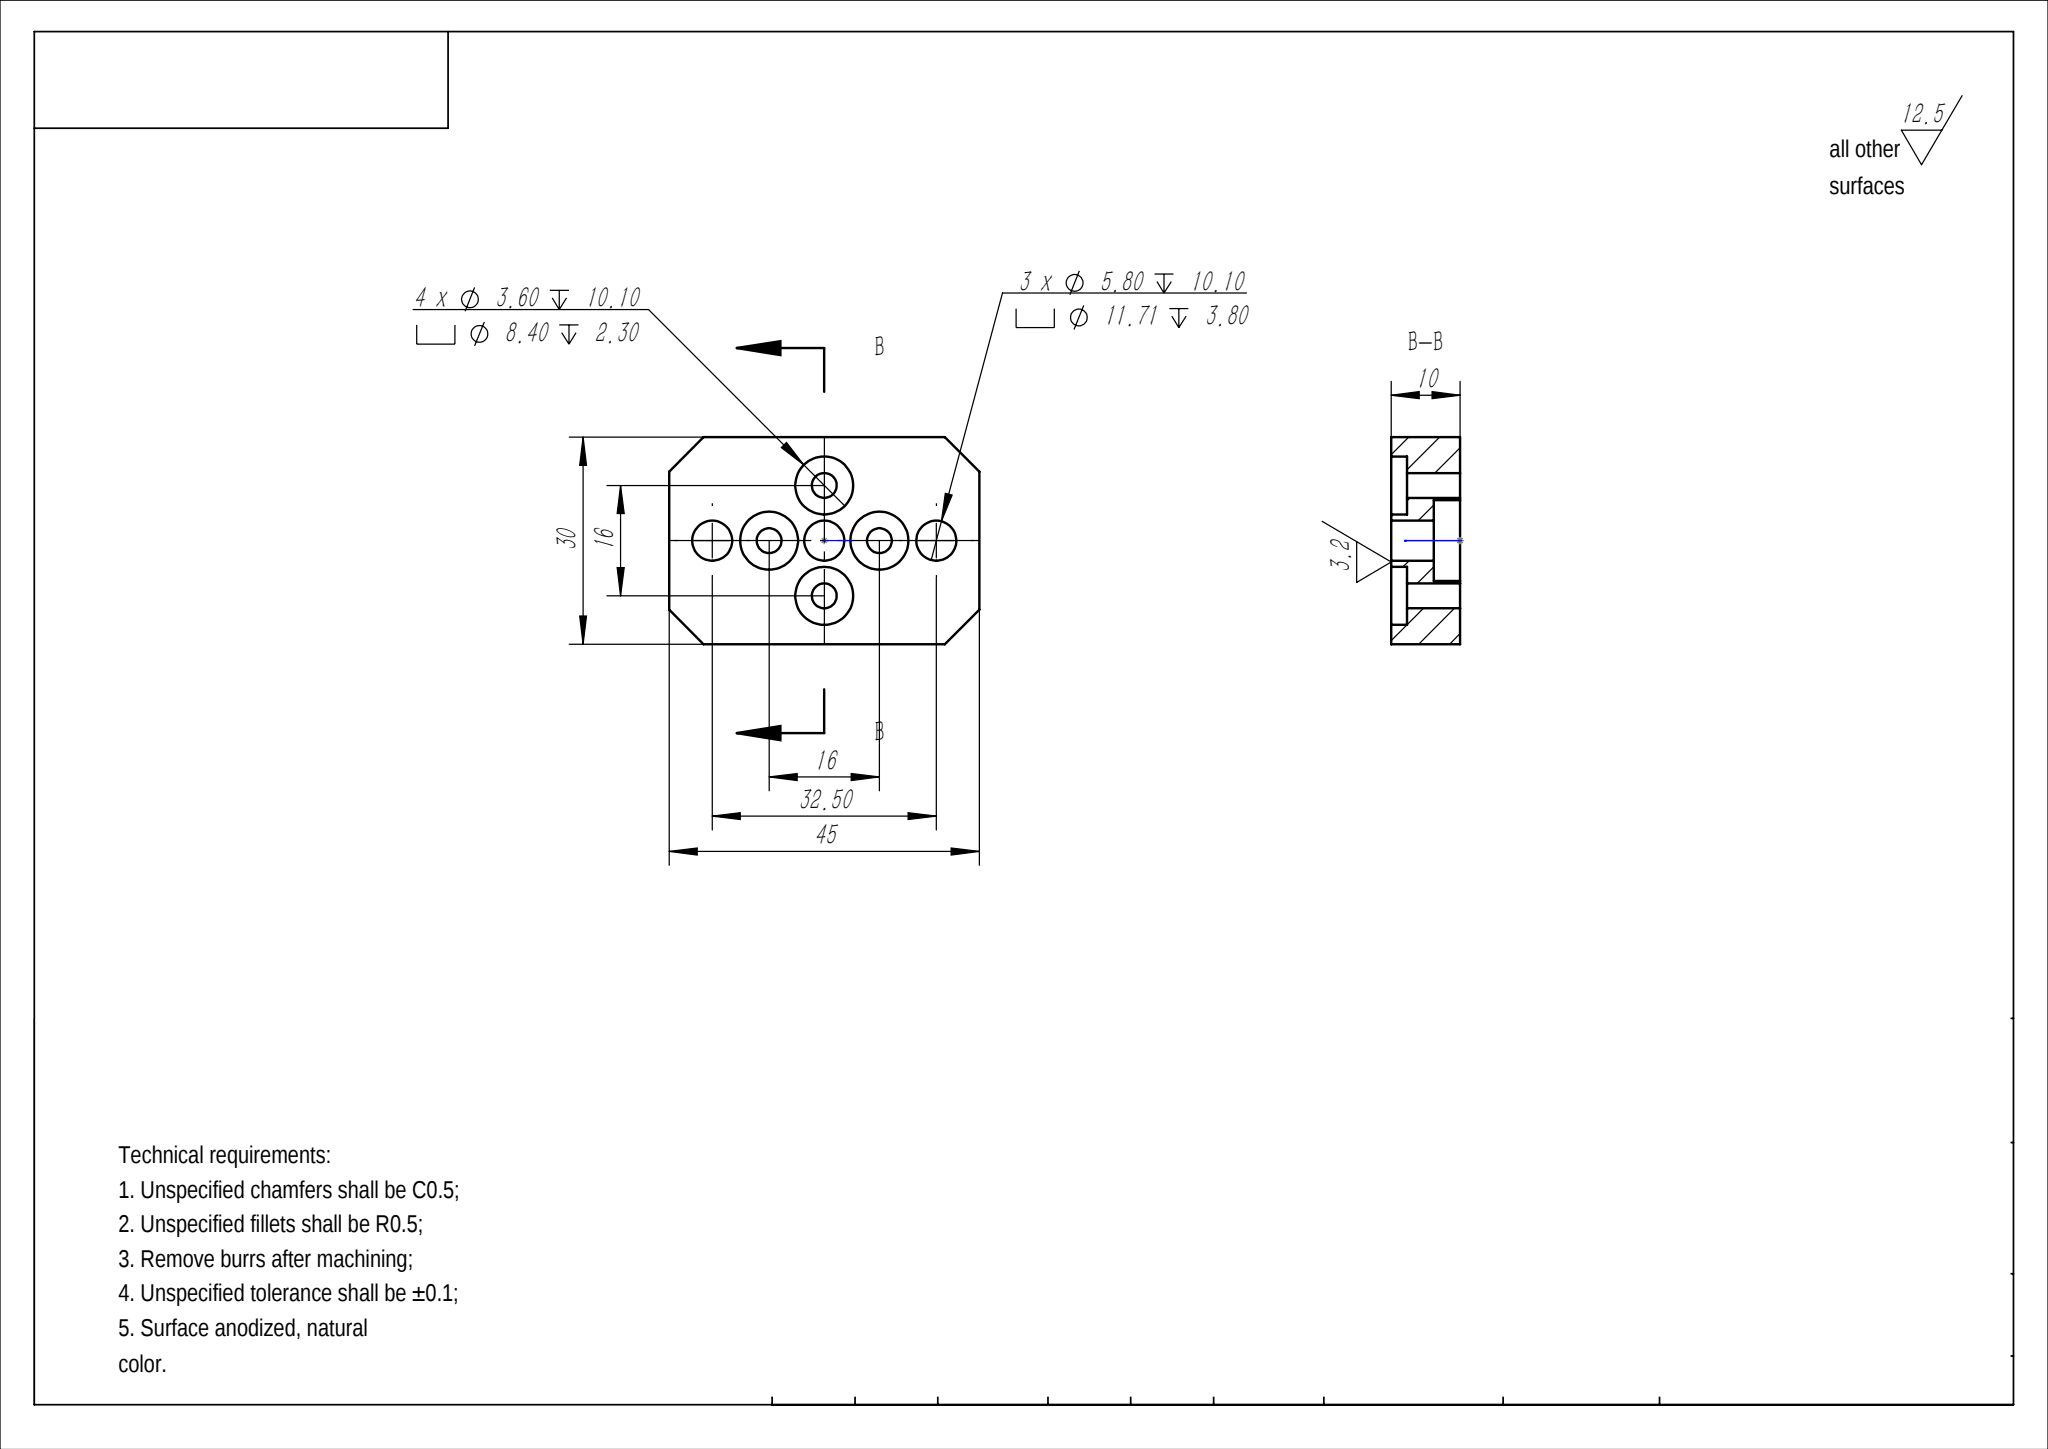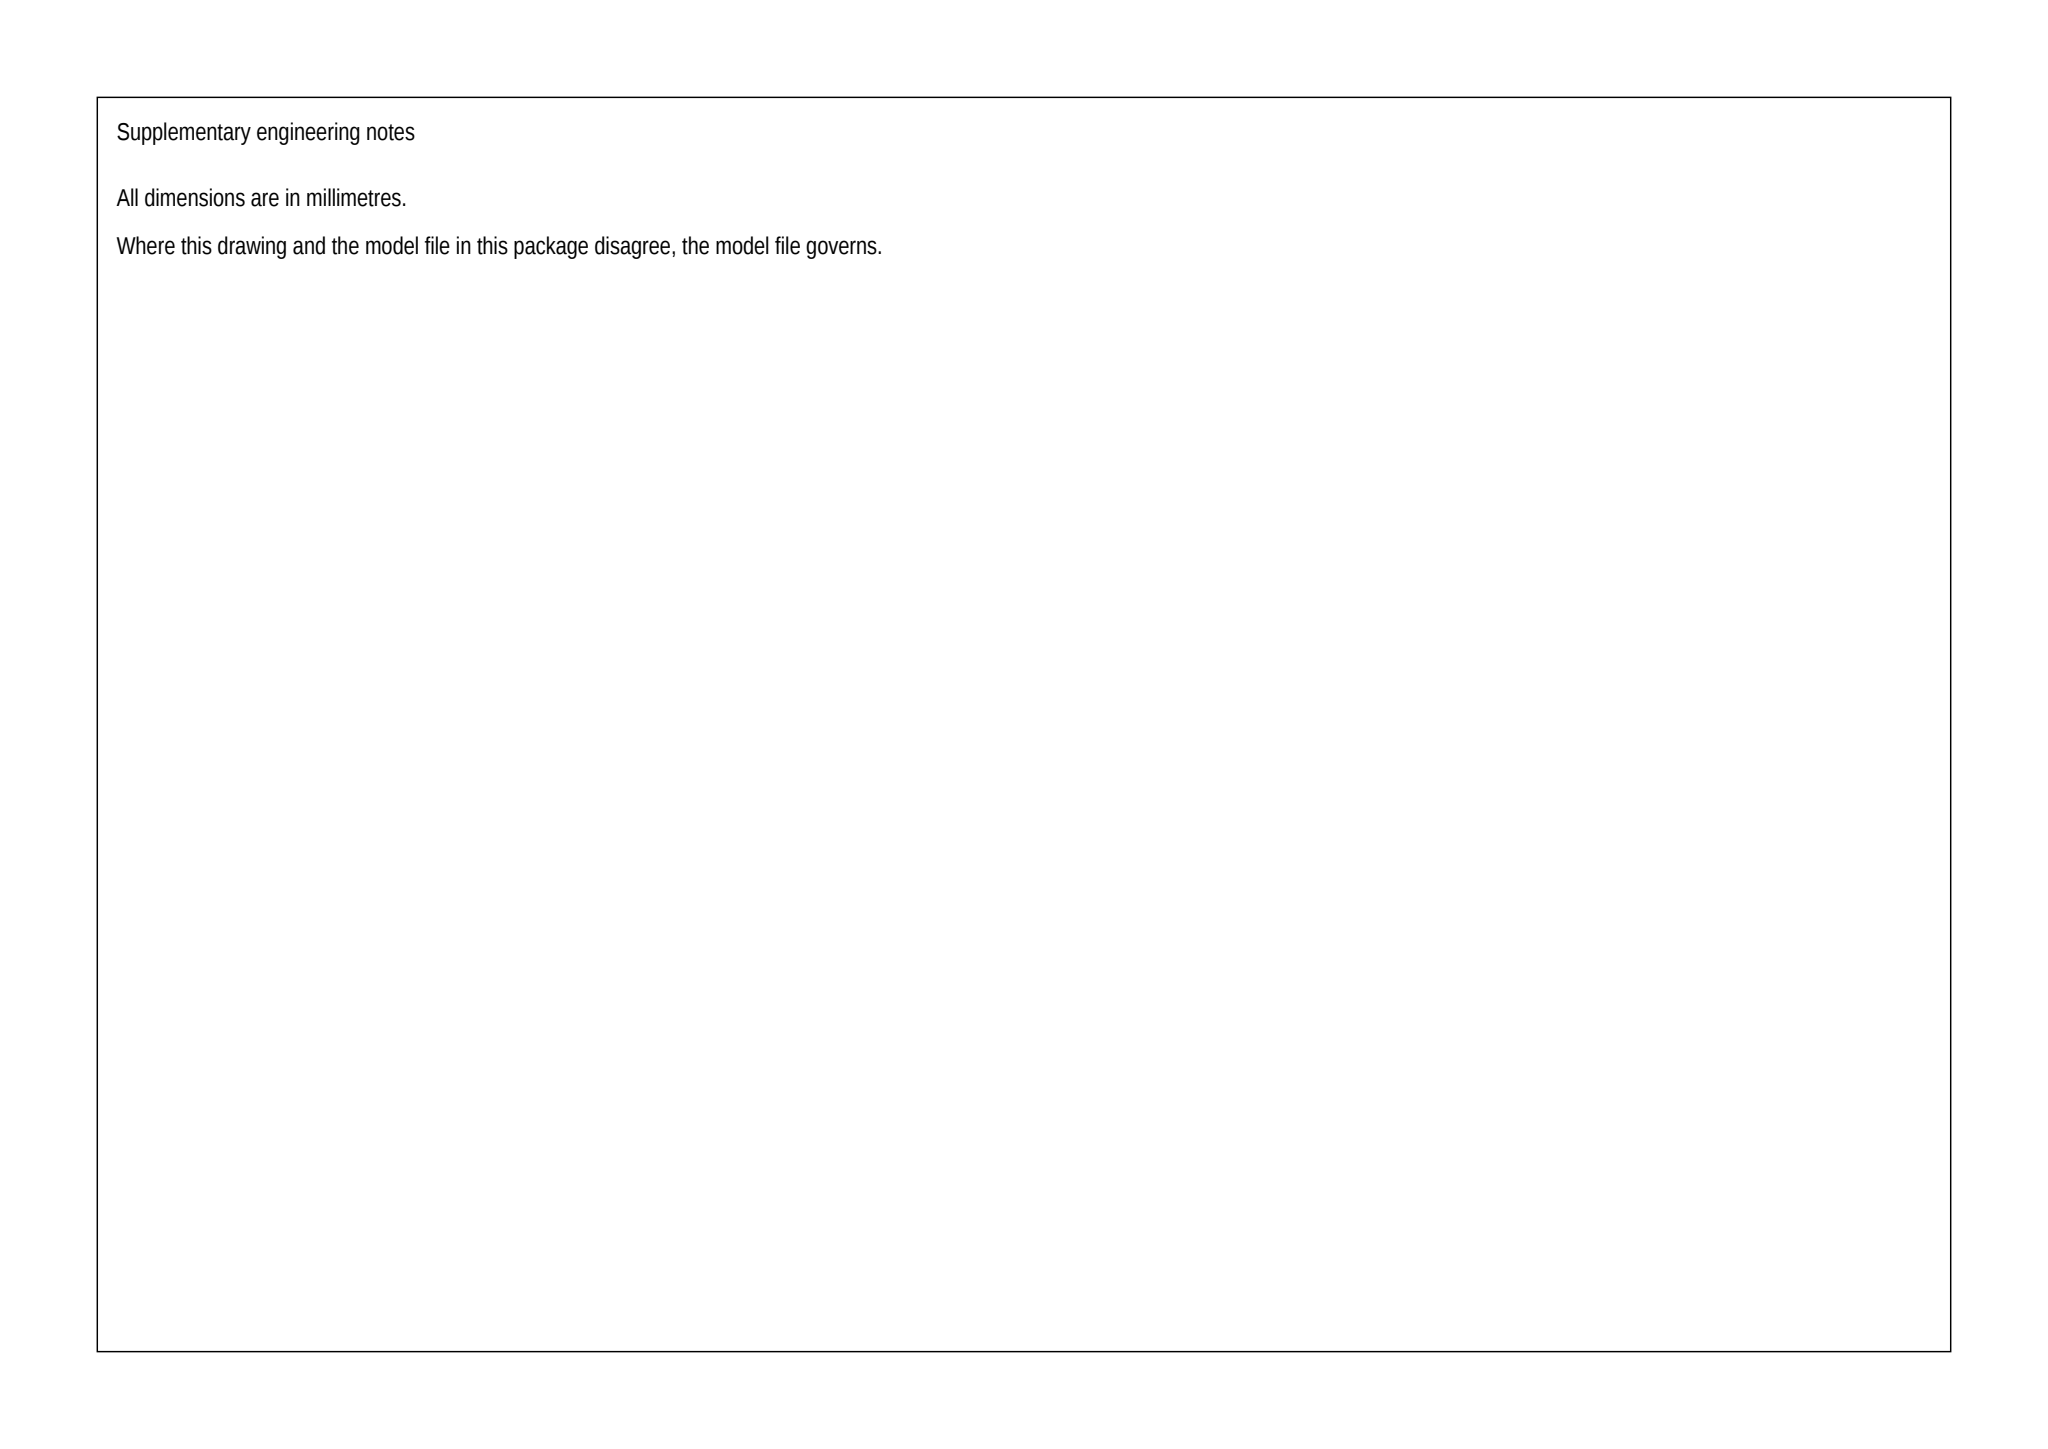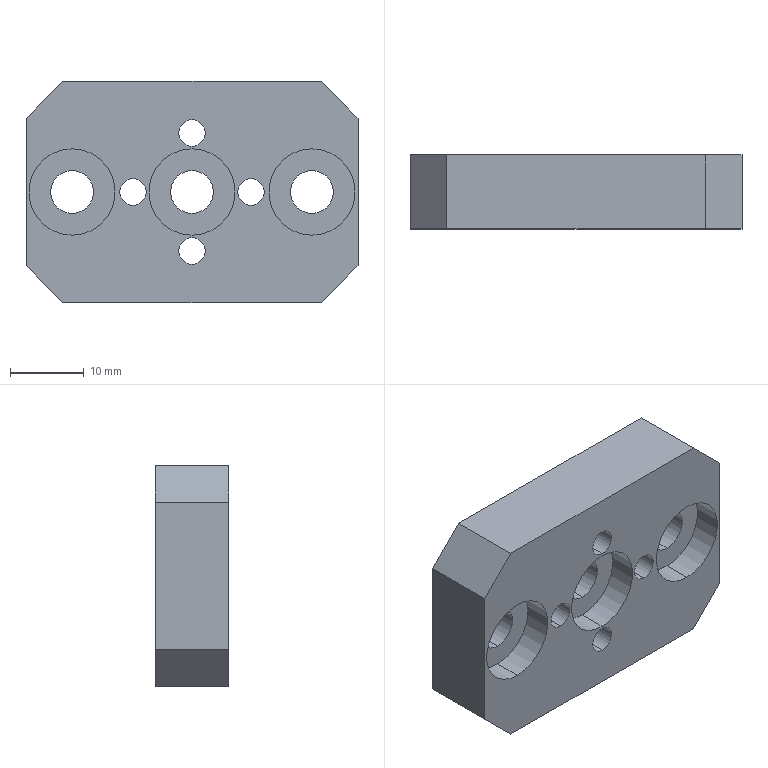Part | SolidWorks | mm | 1 solid | 45 faces | box 45 x 10 x 30 mm | volume 10457 mm3 | cylinder 28 | plane 17 | commonest cylinder face diameters 8.4 x8 3.6 x8 11.71 x6 5.8 x6
build123d program:
from build123d import *

# Parameters (mm, degrees)
SKETCH1_W                                           = 45
SKETCH1_H                                           = 30
BOSS_EXTRUDE1_DEPTH                                 = 10
CYLINDRICAL_COUNTERSUNK_HOLE_FOR_M5_HEX_D           = 5.8
CYLINDRICAL_COUNTERSUNK_HOLE_FOR_M5_HEX_DEPTH       = 10.1
CYLINDRICAL_COUNTERSUNK_HOLE_FOR_M5_HEX_CBORE_D     = 11.71
CYLINDRICAL_COUNTERSUNK_HOLE_FOR_M5_HEX_CBORE_DEPTH = 3.8
CYLINDRICAL_COUNTERSUNK_HOLE_FOR_M5_HEX_TIP         = 1.742
CYLINDRICAL_COUNTERSUNK_HOLE_FOR_M3_HEX_D           = 3.6
CYLINDRICAL_COUNTERSUNK_HOLE_FOR_M3_HEX_DEPTH       = 10.1
CYLINDRICAL_COUNTERSUNK_HOLE_FOR_M3_HEX_CBORE_D     = 8.4
CYLINDRICAL_COUNTERSUNK_HOLE_FOR_M3_HEX_CBORE_DEPTH = 2.3
CYLINDRICAL_COUNTERSUNK_HOLE_FOR_M3_HEX_TIP         = 1.082
CHAMFER1_SIZE                                       = 5


with BuildPart() as part:
    # Sketch1 → Boss-Extrude1 (new body)
    with BuildSketch(Plane(origin=(0, 0, 0), x_dir=(1, 0, 0), z_dir=(0, 1, 0))):
        Rectangle(SKETCH1_W, SKETCH1_H)
    extrude(amount=BOSS_EXTRUDE1_DEPTH)

    # Cylindrical Countersunk Hole for M5 Hex
    with Locations(Plane(origin=(0, 0, 0), x_dir=(-1, 0, 0), z_dir=(0, -1, 0))):
        with Locations((16.25, 0), (0, 0), (-16.25, 0)):
            CounterBoreHole(CYLINDRICAL_COUNTERSUNK_HOLE_FOR_M5_HEX_D / 2, CYLINDRICAL_COUNTERSUNK_HOLE_FOR_M5_HEX_CBORE_D / 2, CYLINDRICAL_COUNTERSUNK_HOLE_FOR_M5_HEX_CBORE_DEPTH, depth=CYLINDRICAL_COUNTERSUNK_HOLE_FOR_M5_HEX_DEPTH)
            with Locations((0, 0, -(CYLINDRICAL_COUNTERSUNK_HOLE_FOR_M5_HEX_DEPTH + CYLINDRICAL_COUNTERSUNK_HOLE_FOR_M5_HEX_TIP / 2))):  # 118° drill point
                Cone(0, CYLINDRICAL_COUNTERSUNK_HOLE_FOR_M5_HEX_D / 2, CYLINDRICAL_COUNTERSUNK_HOLE_FOR_M5_HEX_TIP, mode=Mode.SUBTRACT)

    # Cylindrical Countersunk Hole for M3 Hex
    with Locations(Plane(origin=(0, 10, 0), x_dir=(1, 0, 0), z_dir=(0, 1, 0))):
        with Locations((0, 8), (8, 0), (0, -8), (-8, 0)):
            CounterBoreHole(CYLINDRICAL_COUNTERSUNK_HOLE_FOR_M3_HEX_D / 2, CYLINDRICAL_COUNTERSUNK_HOLE_FOR_M3_HEX_CBORE_D / 2, CYLINDRICAL_COUNTERSUNK_HOLE_FOR_M3_HEX_CBORE_DEPTH, depth=CYLINDRICAL_COUNTERSUNK_HOLE_FOR_M3_HEX_DEPTH)
            with Locations((0, 0, -(CYLINDRICAL_COUNTERSUNK_HOLE_FOR_M3_HEX_DEPTH + CYLINDRICAL_COUNTERSUNK_HOLE_FOR_M3_HEX_TIP / 2))):  # 118° drill point
                Cone(0, CYLINDRICAL_COUNTERSUNK_HOLE_FOR_M3_HEX_D / 2, CYLINDRICAL_COUNTERSUNK_HOLE_FOR_M3_HEX_TIP, mode=Mode.SUBTRACT)

    # Chamfer1
    chamfer1_edges = [part.edges().sort_by_distance(p)[0] for p in [
        (22.5, 5, 15),
        (-22.5, 5, 15),
        (-22.5, 5, -15),
        (22.5, 5, -15),
    ]]
    chamfer(chamfer1_edges, length=CHAMFER1_SIZE)


solid = part.part